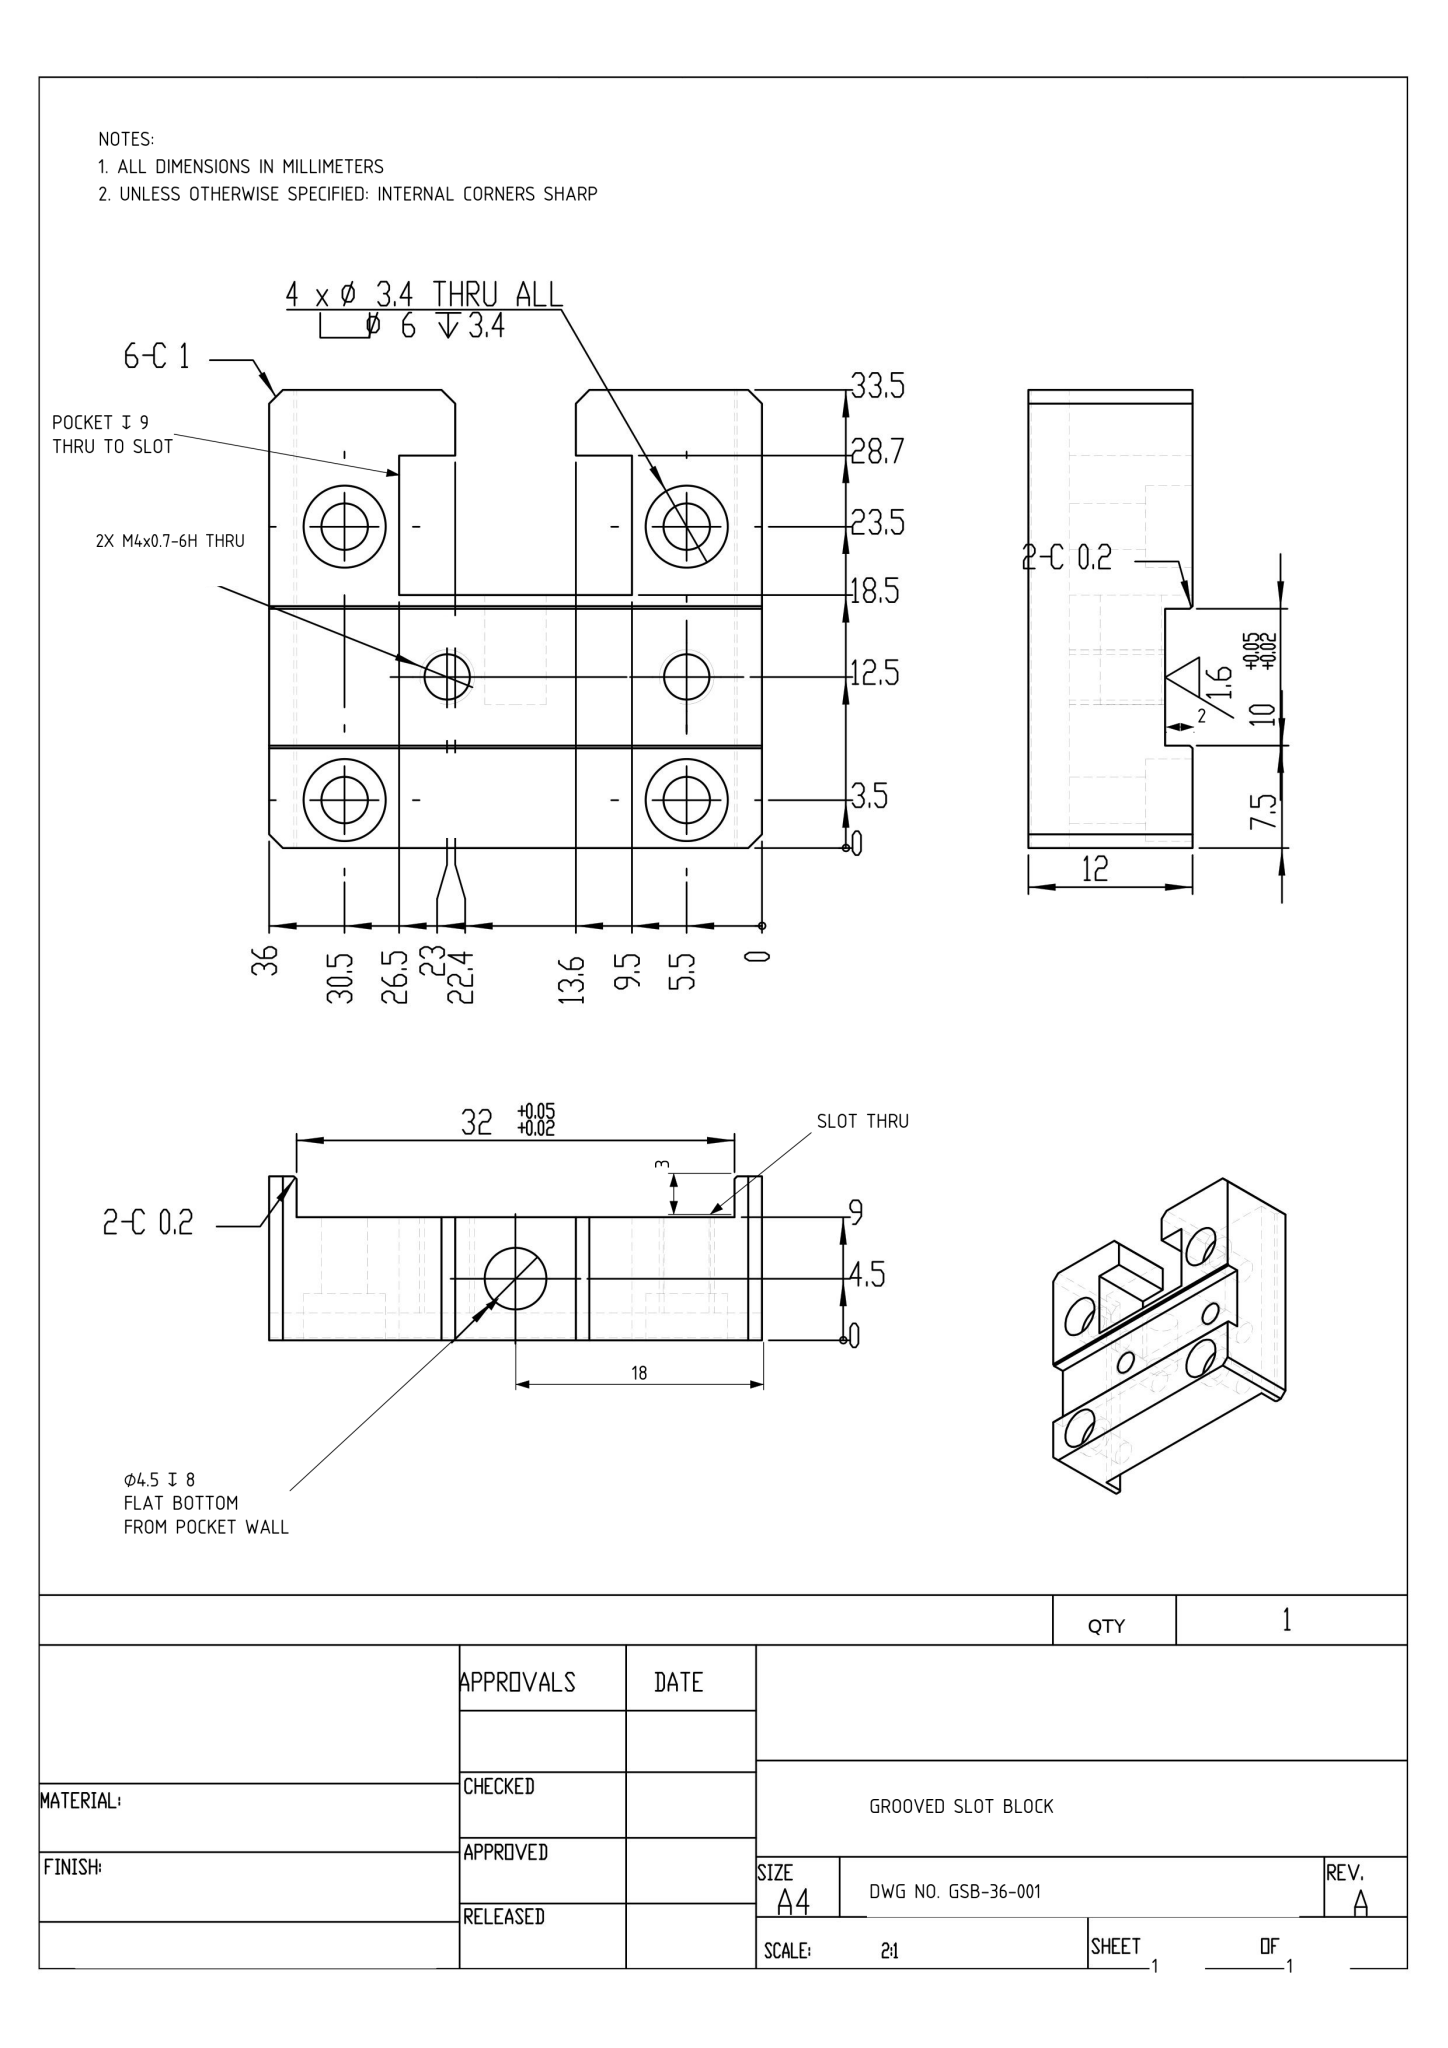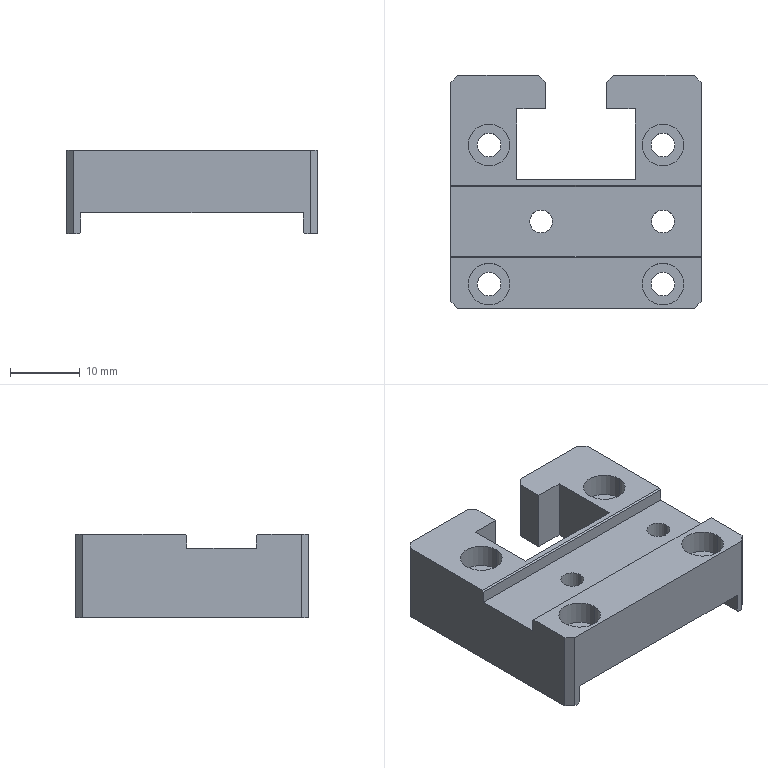Part | NX | mm | 1 solid | 59 faces | box 36 x 33.5 x 12 mm | volume 7725 mm3 | plane 37 | cylinder 22 | commonest cylinder face diameters 3.4 x8 6 x8 3.3 x4 4.5 x2